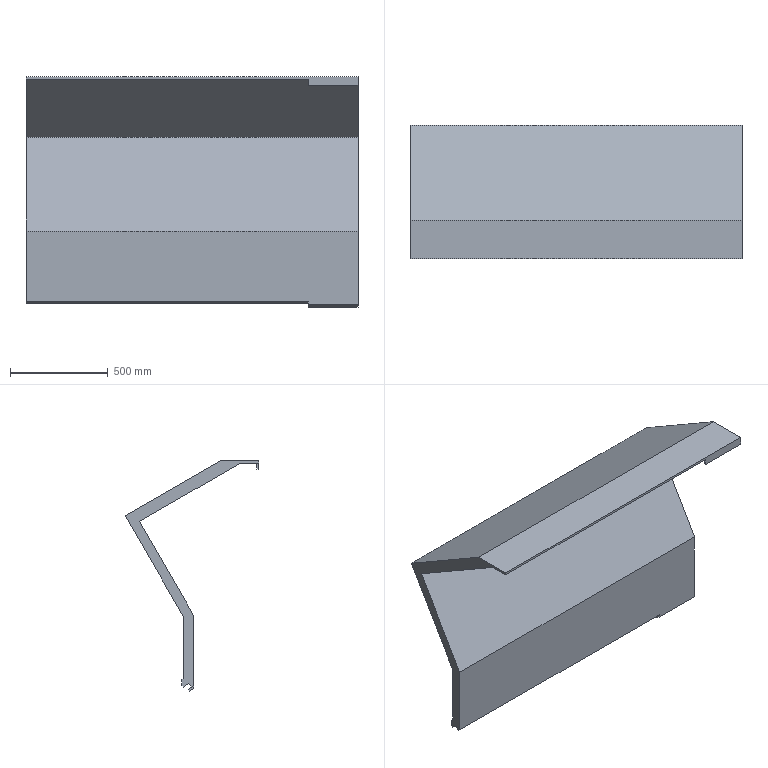Component | NX | SIM15_ABEDECKUNG_OBEN_LINKS_NEU | 1 solid | 26 faces | volume 142778714 mm3 | plane 26